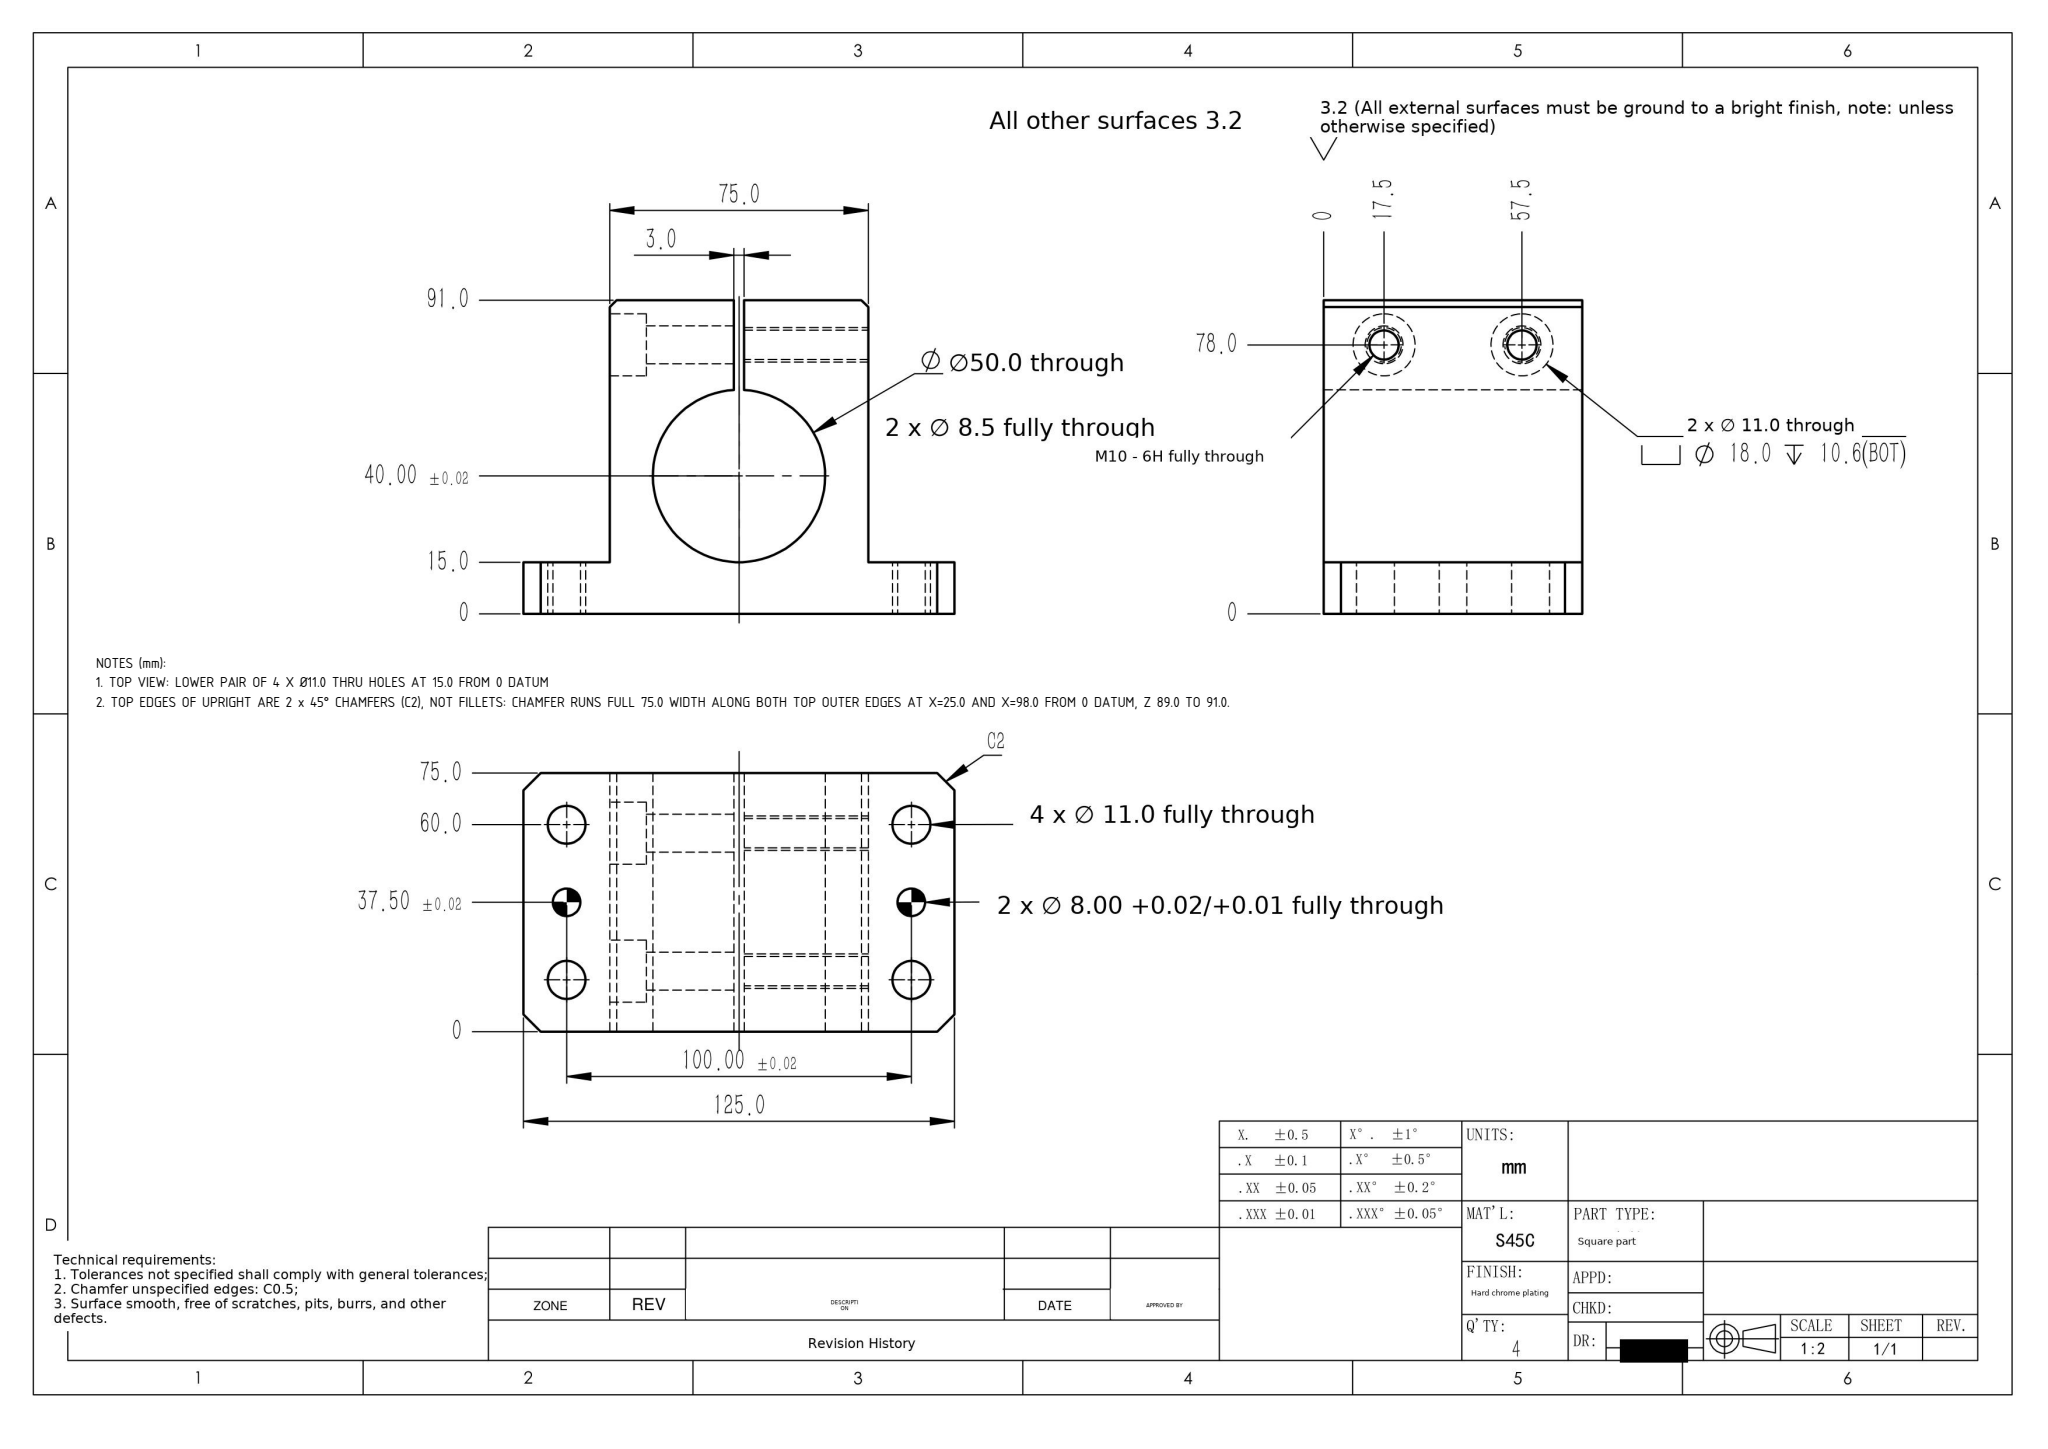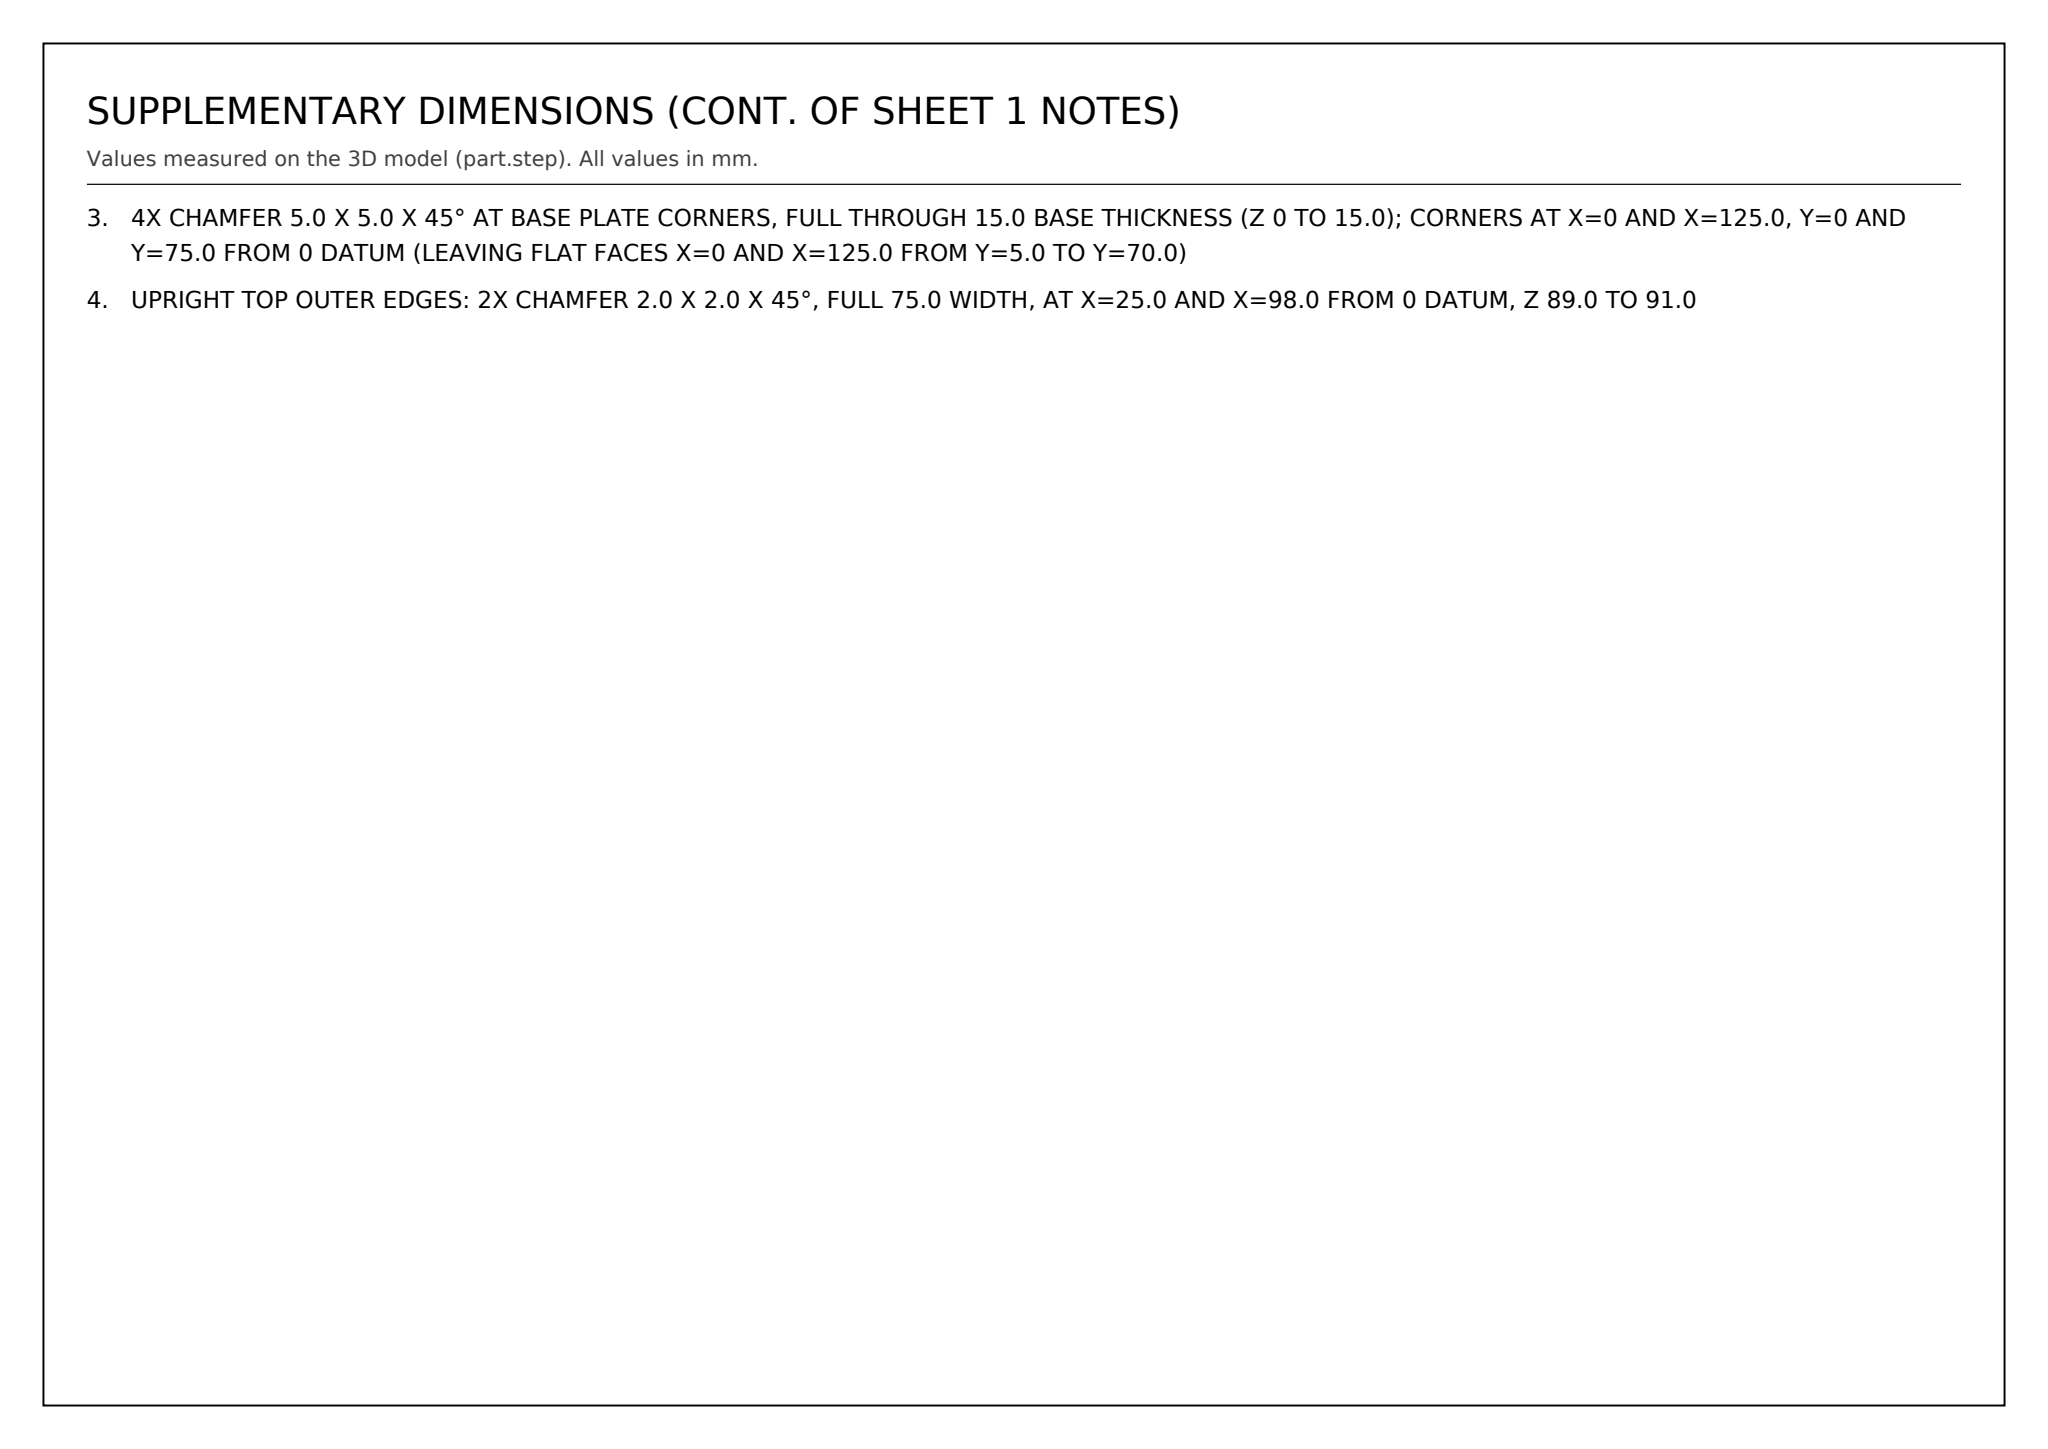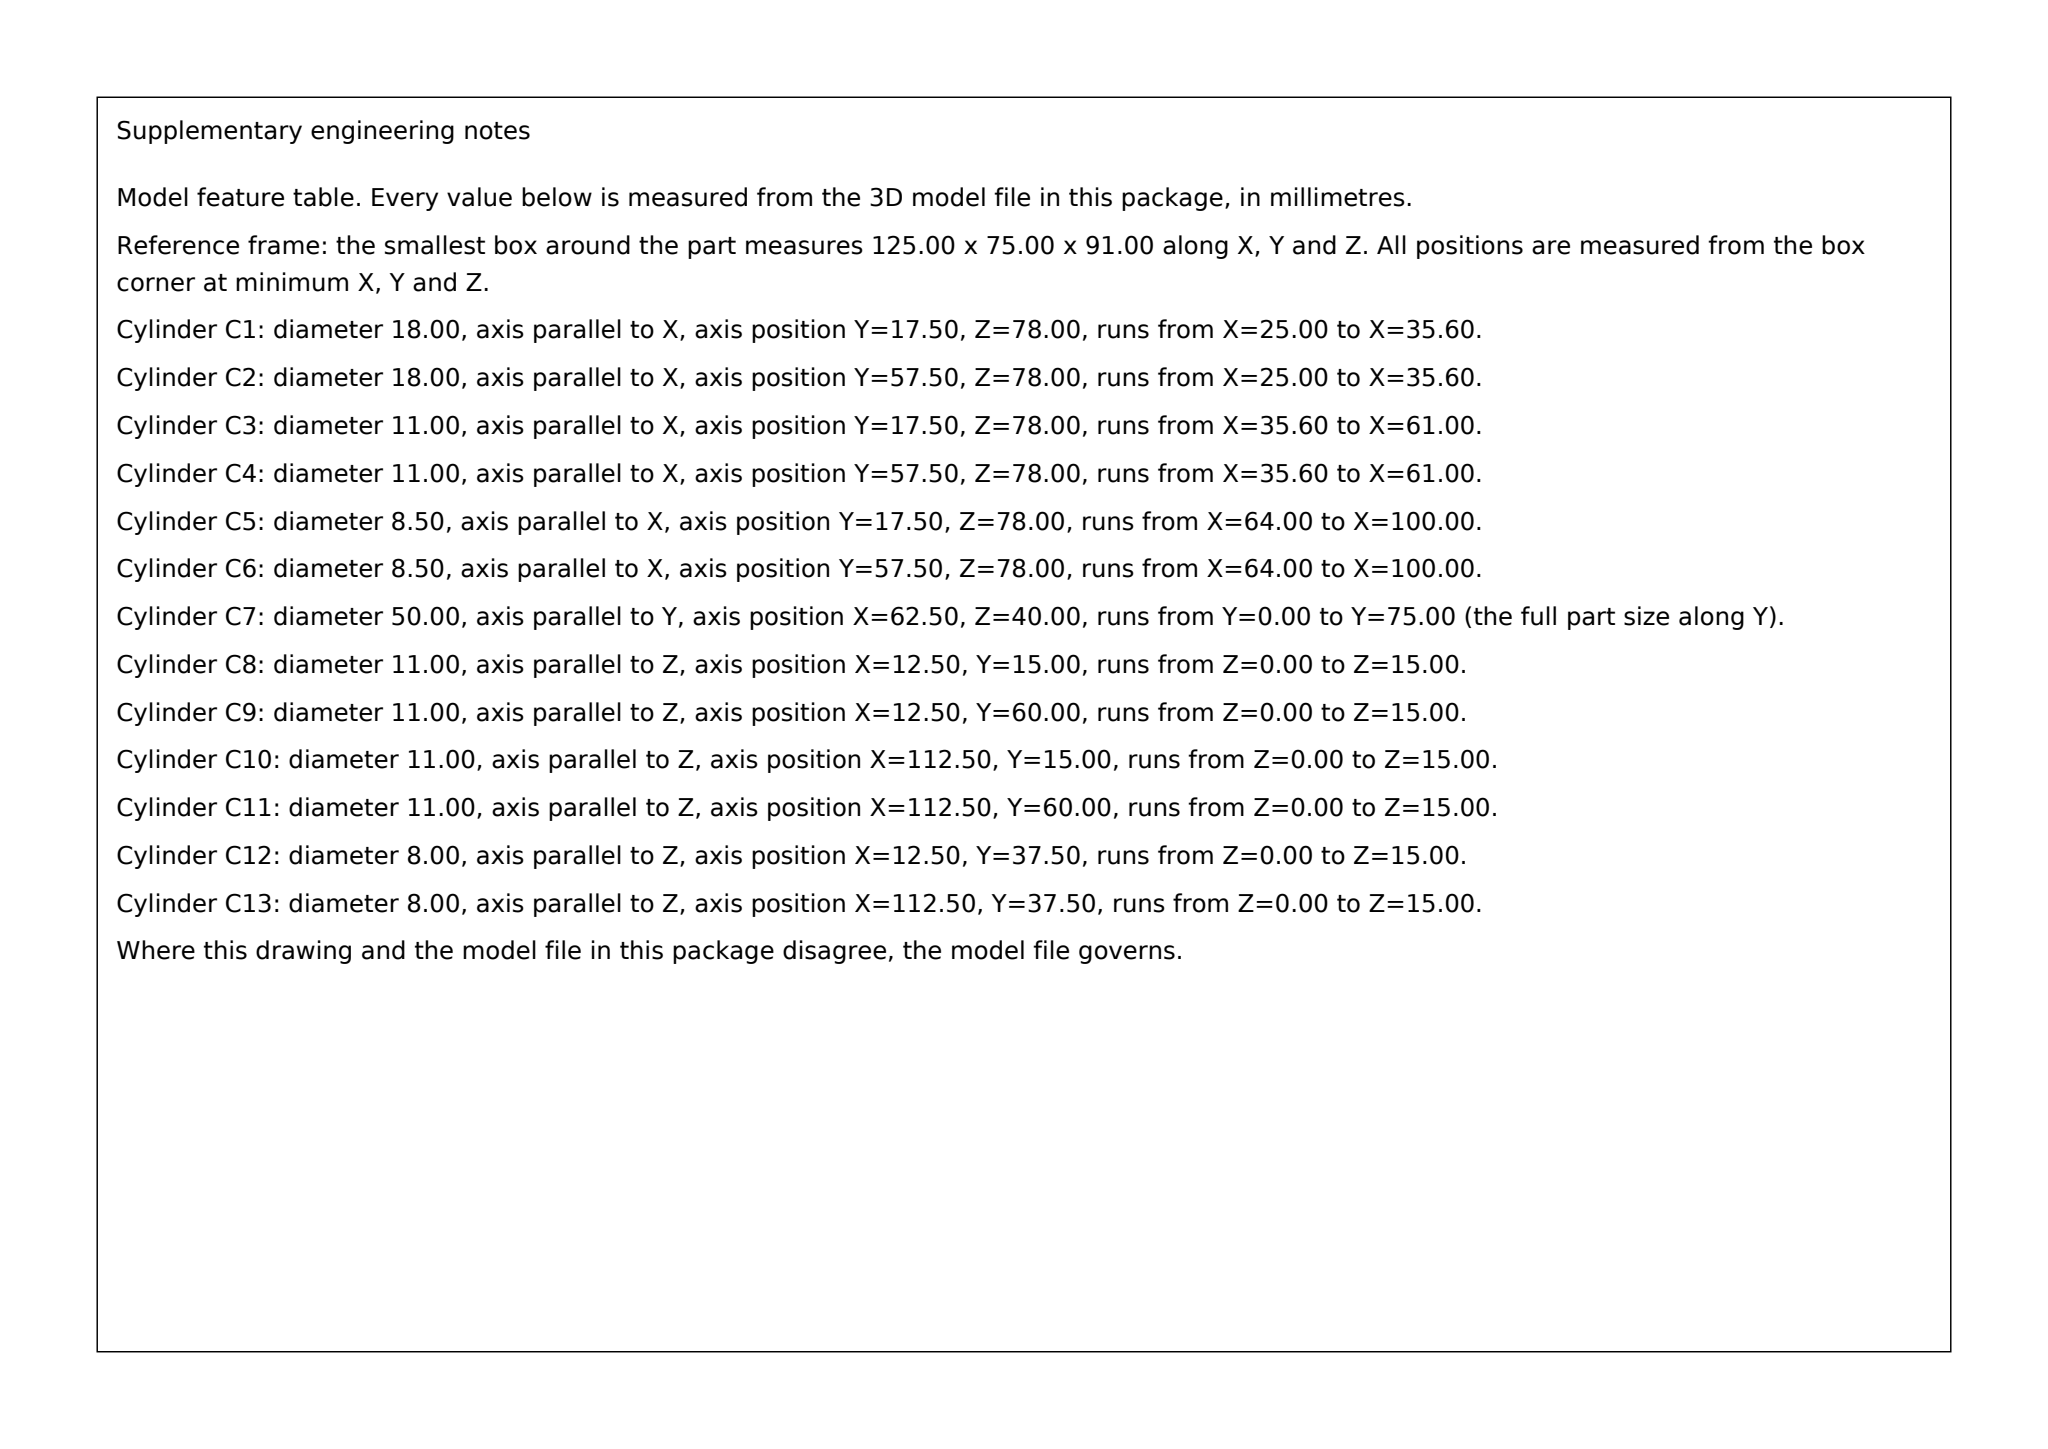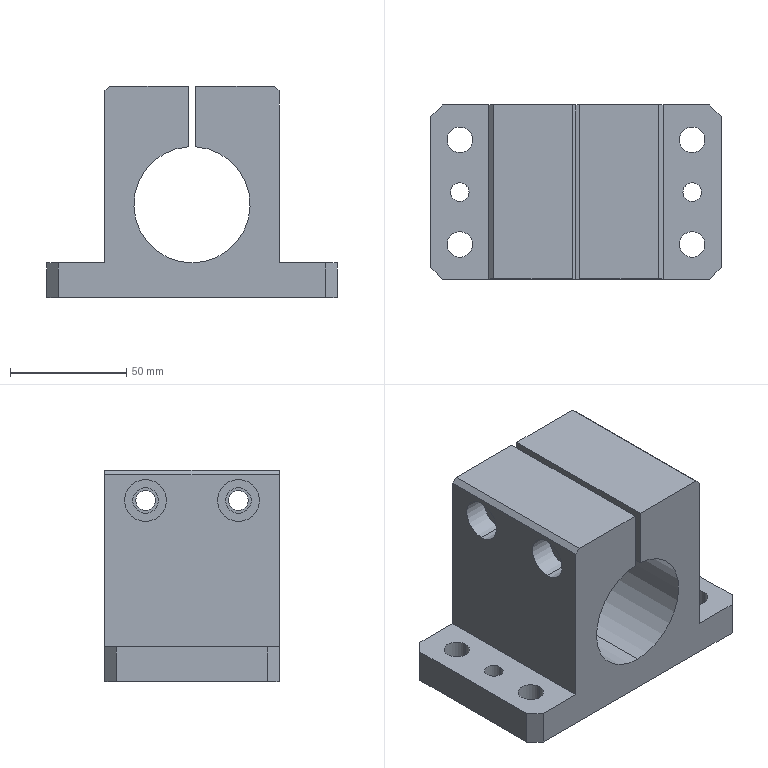Part | SolidWorks | mm | 1 solid | 47 faces | box 125 x 75 x 91 mm | volume 392441 mm3 | cylinder 26 | plane 21 | commonest cylinder face diameters 11 x12 8 x4 8.5 x4 18 x4 50 x2
Drawing notes:
TOP VIEW: LOWER PAIR OF 4 X Ø11.0 THRU HOLES AT 15.0 FROM 0 DATUM | from the solid: Cylinders Ø11.0 axis z at (12.5,15.0) and (112.5,15.0), L=15.0; upper pair at y=60.0, bbox y 0-75
TOP EDGES OF UPRIGHT ARE 2 x 45° CHAMFERS (C2), NOT FILLETS: CHAMFER RUNS FULL 75.0 WIDTH ALONG BOTH TOP OUTER EDGES AT X=25.0 AND X=98.0 FROM 0 DATUM, Z 89.0 TO 91.0. | from the solid: inclined_planes: two faces angle_to_xyz_axes [45,90,45], bbox_from [25.0,0,89.0] and [98.0,0,89.0], size [2.0,75.0,2.0]; tori list is empty (no blend radii present)
4X CHAMFER 5.0 X 5.0 X 45° AT BASE PLATE CORNERS, FULL THROUGH 15.0 BASE THICKNESS (Z 0 TO 15.0); CORNERS AT X=0 AND X=125.0, Y=0 AND Y=75.0 FROM 0 DATUM (LEAVING FLAT FACES X=0 AND X=125.0 FROM Y=5.0 TO Y=70.0) | from the solid: inclined_planes: four faces angle_to_xyz_axes [45,45,90], size [5.0,5.0,15.0] at bbox_from [0,0,0], [0,70,0], [120,0,0], [120,70,0]; axis_planes x=0 and x=125.0 with y extent [5.0,70.0], z [0,15.0]
UPRIGHT TOP OUTER EDGES: 2X CHAMFER 2.0 X 2.0 X 45°, FULL 75.0 WIDTH, AT X=25.0 AND X=98.0 FROM 0 DATUM, Z 89.0 TO 91.0 | from the solid: inclined_planes: angle_to_xyz_axes [45,90,45], size [2.0,75.0,2.0] at bbox_from [25.0,0,89.0] and [98.0,0,89.0]
build123d program:
from build123d import *

# Parameters (mm, degrees)
SKETCH1_W                                        = 125
SKETCH1_H                                        = 75
BOSS_EXTRUDE1_DEPTH                              = 91
SKETCH2_W                                        = 25
SKETCH2_H                                        = 76
CUT_EXTRUDE1_DEPTH                               = 134.463
SKETCH3_R                                        = 25
CUT_EXTRUDE2_DEPTH                               = 134.463
SKETCH4_W                                        = 3
SKETCH4_H                                        = 33
CUT_EXTRUDE3_DEPTH                               = 134.463
M10_HEX_SOCKET_HEAD_CAP_SCREW_CBORE1_D           = 11
M10_HEX_SOCKET_HEAD_CAP_SCREW_CBORE1_DEPTH       = 36
M10_HEX_SOCKET_HEAD_CAP_SCREW_CBORE1_CBORE_D     = 18
M10_HEX_SOCKET_HEAD_CAP_SCREW_CBORE1_CBORE_DEPTH = 10.6
M10_TAPPED_HOLE1_D                               = 8.5
M10_CLEARANCE_HOLE1_D                            = 11
SIZE_MM_DOWEL_PIN_HOLE1_D                        = 8
CHAMFER1_SIZE                                    = 5
CHAMFER2_SIZE                                    = 2


with BuildPart() as part:
    # Sketch1 → Boss-Extrude1 (new body)
    with BuildSketch(Plane.XY):
        Rectangle(SKETCH1_W, SKETCH1_H)
    extrude(amount=BOSS_EXTRUDE1_DEPTH)

    # Sketch2 → Cut-Extrude1 (cut, through all)
    with BuildSketch(Plane(origin=(0, 37.5, 0), x_dir=(1, 0, 0), z_dir=(0, 1, 0))):
        with Locations((-50, -53)):
            Rectangle(SKETCH2_W, SKETCH2_H)
        with Locations((50, -53)):
            Rectangle(SKETCH2_W, SKETCH2_H)
    extrude(amount=-CUT_EXTRUDE1_DEPTH, mode=Mode.SUBTRACT)

    # Sketch3 → Cut-Extrude2 (cut, through all)
    with BuildSketch(Plane.XZ.offset(37.5)):
        with Locations(Location((0, 40, 0), (0, 0, 270))):
            Circle(SKETCH3_R)
    extrude(amount=-CUT_EXTRUDE2_DEPTH, mode=Mode.SUBTRACT)

    # Sketch4 → Cut-Extrude3 (cut, through all)
    with BuildSketch(Plane.XZ.offset(37.5)):
        with Locations((0, 76.5)):
            Rectangle(SKETCH4_W, SKETCH4_H)
    extrude(amount=-CUT_EXTRUDE3_DEPTH, mode=Mode.SUBTRACT)

    # M10 Hex Socket Head Cap Screw CBORE1
    with Locations(Plane.ZY.offset(37.5)):
        with Locations((78, 20), (78, -20)):
            CounterBoreHole(M10_HEX_SOCKET_HEAD_CAP_SCREW_CBORE1_D / 2, M10_HEX_SOCKET_HEAD_CAP_SCREW_CBORE1_CBORE_D / 2, M10_HEX_SOCKET_HEAD_CAP_SCREW_CBORE1_CBORE_DEPTH, depth=M10_HEX_SOCKET_HEAD_CAP_SCREW_CBORE1_DEPTH)

    # M10 Tapped Hole1 (through all)
    with Locations(Plane.ZY.offset(-1.5)):
        with Locations((78, 20), (78, -20)):
            Hole(M10_TAPPED_HOLE1_D / 2)

    # M10 Clearance Hole1 (through all)
    with Locations(Plane.XY.offset(15)):
        with Locations((50, 22.5), (50, -22.5), (-50, -22.5), (-50, 22.5)):
            Hole(M10_CLEARANCE_HOLE1_D / 2)

    # Size mm Dowel Pin Hole1 (through all)
    with Locations(Plane.XY.offset(15)):
        with Locations((-50, 0), (50, 0)):
            Hole(SIZE_MM_DOWEL_PIN_HOLE1_D / 2)

    # Chamfer1
    chamfer1_edges = [part.edges().sort_by_distance(p)[0] for p in [
        (-62.5, -37.5, 7.5),
        (-62.5, 37.5, 7.5),
        (62.5, -37.5, 7.5),
        (62.5, 37.5, 7.5),
    ]]
    chamfer(chamfer1_edges, length=CHAMFER1_SIZE)

    # Chamfer2
    chamfer2_edges = [part.edges().sort_by_distance(p)[0] for p in [
        (-37.5, 0, 91),
        (37.5, 0, 91),
    ]]
    chamfer(chamfer2_edges, length=CHAMFER2_SIZE)


solid = part.part